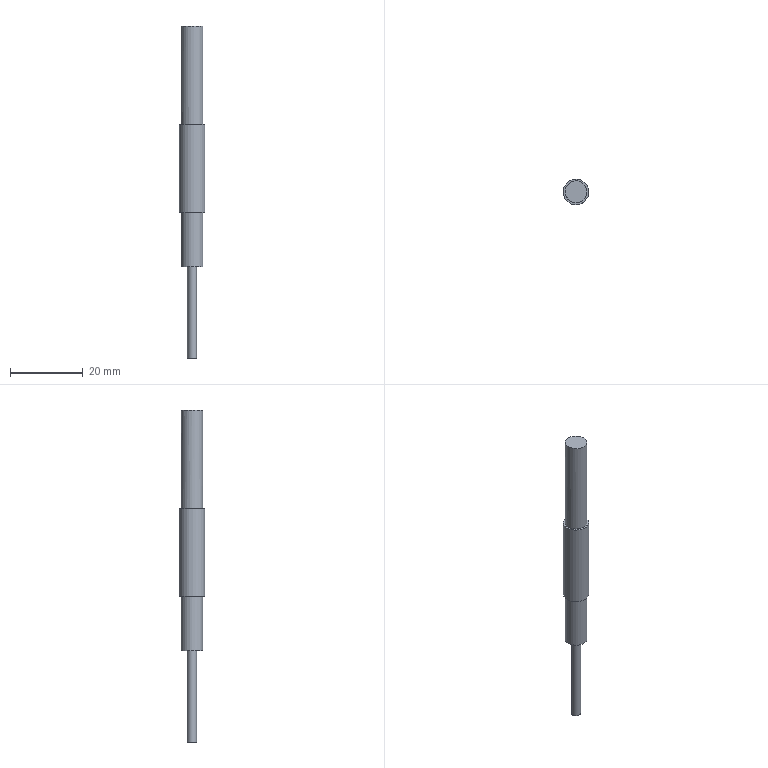Component | NX | DRIVE_SHAFT | 1 solid | 9 faces | box 7 x 7 x 91 mm | volume 2234 mm3 | plane 5 | cylinder 4 | commonest cylinder face diameters 6 x2 7 x1 2.5 x1
STEP:
#1=CARTESIAN_POINT('',(0.,0.,0.));
#2=DIRECTION('',(0.,0.,1.));
#3=DIRECTION('',(1.,0.,0.));
#4=AXIS2_PLACEMENT_3D('',#1,#2,#3);
#5=CARTESIAN_POINT('',(-3.16,-2.811,44.));
#6=VERTEX_POINT('',#5);
#7=CARTESIAN_POINT('',(-5.267,-0.01624,44.));
#8=DIRECTION('',(0.,0.,1.));
#9=DIRECTION('',(0.6018,-0.7986,0.));
#10=AXIS2_PLACEMENT_3D('',#7,#8,#9);
#11=CIRCLE('',#10,3.5);
#12=CARTESIAN_POINT('',(-2.871,1.789,44.));
#13=DIRECTION('',(0.,0.,1.));
#14=DIRECTION('',(0.6018,-0.7986,0.));
#15=AXIS2_PLACEMENT_3D('',#12,#13,#14);
#16=PLANE('',#15);
#17=CARTESIAN_POINT('',(0.,-3.));
#18=DIRECTION('',(1.,0.));
#19=AXIS2_PLACEMENT_2D('',#17,#18);
#20=CIRCLE('',#19,3.5);
#21=(GEOMETRIC_REPRESENTATION_CONTEXT(2)PARAMETRIC_REPRESENTATION_CONTEXT()REPRESENTATION_CONTEXT('',''));
#22=DEFINITIONAL_REPRESENTATION('',(#20),#21);
#23=PCURVE('',#16,#22);
#24=CARTESIAN_POINT('',(-5.267,-0.01624,56.));
#25=DIRECTION('',(0.,0.,1.));
#26=DIRECTION('',(0.6018,-0.7986,0.));
#27=AXIS2_PLACEMENT_3D('',#24,#25,#26);
#28=CYLINDRICAL_SURFACE('',#27,3.5);
#29=CARTESIAN_POINT('',(0.,-12.));
#30=DIRECTION('',(1.,0.));
#31=VECTOR('',#30,1.);
#32=LINE('',#29,#31);
#33=(GEOMETRIC_REPRESENTATION_CONTEXT(2)PARAMETRIC_REPRESENTATION_CONTEXT()REPRESENTATION_CONTEXT('',''));
#34=DEFINITIONAL_REPRESENTATION('',(#32),#33);
#35=PCURVE('',#28,#34);
#36=SURFACE_CURVE('',#11,(#23,#35),.PCURVE_S1.);
#37=EDGE_CURVE('',#6,#6,#36,.T.);
#38=ORIENTED_EDGE('',*,*,#37,.T.);
#39=EDGE_LOOP('',(#38));
#40=FACE_BOUND('',#39,.T.);
#41=CARTESIAN_POINT('',(-3.461,-2.412,44.));
#42=VERTEX_POINT('',#41);
#43=CARTESIAN_POINT('',(-5.267,-0.01624,44.));
#44=DIRECTION('',(0.,0.,1.));
#45=DIRECTION('',(0.6018,-0.7986,0.));
#46=AXIS2_PLACEMENT_3D('',#43,#44,#45);
#47=CIRCLE('',#46,3.);
#48=CARTESIAN_POINT('',(0.,-3.));
#49=DIRECTION('',(1.,0.));
#50=AXIS2_PLACEMENT_2D('',#48,#49);
#51=CIRCLE('',#50,3.);
#52=(GEOMETRIC_REPRESENTATION_CONTEXT(2)PARAMETRIC_REPRESENTATION_CONTEXT()REPRESENTATION_CONTEXT('',''));
#53=DEFINITIONAL_REPRESENTATION('',(#51),#52);
#54=PCURVE('',#16,#53);
#55=CARTESIAN_POINT('',(-5.267,-0.01624,56.));
#56=DIRECTION('',(0.,0.,1.));
#57=DIRECTION('',(0.6018,-0.7986,0.));
#58=AXIS2_PLACEMENT_3D('',#55,#56,#57);
#59=CYLINDRICAL_SURFACE('',#58,3.);
#60=CARTESIAN_POINT('',(0.,-12.));
#61=DIRECTION('',(1.,0.));
#62=VECTOR('',#61,1.);
#63=LINE('',#60,#62);
#64=(GEOMETRIC_REPRESENTATION_CONTEXT(2)PARAMETRIC_REPRESENTATION_CONTEXT()REPRESENTATION_CONTEXT('',''));
#65=DEFINITIONAL_REPRESENTATION('',(#63),#64);
#66=PCURVE('',#59,#65);
#67=SURFACE_CURVE('',#47,(#54,#66),.PCURVE_S1.);
#68=EDGE_CURVE('',#42,#42,#67,.T.);
#69=ORIENTED_EDGE('',*,*,#68,.F.);
#70=EDGE_LOOP('',(#69));
#71=FACE_BOUND('',#70,.T.);
#72=ADVANCED_FACE('',(#40,#71),#16,.T.);
#73=CARTESIAN_POINT('',(-3.16,-2.811,20.));
#74=VERTEX_POINT('',#73);
#75=CARTESIAN_POINT('',(-5.267,-0.01624,20.));
#76=DIRECTION('',(0.,0.,1.));
#77=DIRECTION('',(0.6018,-0.7986,0.));
#78=AXIS2_PLACEMENT_3D('',#75,#76,#77);
#79=CIRCLE('',#78,3.5);
#80=CARTESIAN_POINT('',(0.,-36.));
#81=DIRECTION('',(1.,0.));
#82=VECTOR('',#81,1.);
#83=LINE('',#80,#82);
#84=(GEOMETRIC_REPRESENTATION_CONTEXT(2)PARAMETRIC_REPRESENTATION_CONTEXT()REPRESENTATION_CONTEXT('',''));
#85=DEFINITIONAL_REPRESENTATION('',(#83),#84);
#86=PCURVE('',#28,#85);
#87=CARTESIAN_POINT('',(-2.472,2.09,20.));
#88=DIRECTION('',(0.,0.,-1.));
#89=DIRECTION('',(-0.6018,0.7986,0.));
#90=AXIS2_PLACEMENT_3D('',#87,#88,#89);
#91=PLANE('',#90);
#92=CARTESIAN_POINT('',(-3.5,-3.5));
#93=CARTESIAN_POINT('',(-3.5,2.562));
#94=CARTESIAN_POINT('',(1.75,-0.4689));
#95=CARTESIAN_POINT('',(7.,-3.5));
#96=CARTESIAN_POINT('',(1.75,-6.531));
#97=CARTESIAN_POINT('',(-3.5,-9.562));
#98=CARTESIAN_POINT('',(-3.5,-3.5));
#99=(BOUNDED_CURVE()B_SPLINE_CURVE(2,(#92,#93,#94,#95,#96,#97,#98),.UNSPECIFIED.,.T.,.F.)B_SPLINE_CURVE_WITH_KNOTS((1,2,2,2,2,1),(-2.094,0.,2.094,4.189,6.283,8.378),.UNSPECIFIED.)CURVE()GEOMETRIC_REPRESENTATION_ITEM()RATIONAL_B_SPLINE_CURVE((1.,0.5,1.,0.5,1.,0.5,1.))REPRESENTATION_ITEM(''));
#100=(GEOMETRIC_REPRESENTATION_CONTEXT(2)PARAMETRIC_REPRESENTATION_CONTEXT()REPRESENTATION_CONTEXT('',''));
#101=DEFINITIONAL_REPRESENTATION('',(#99),#100);
#102=PCURVE('',#91,#101);
#103=SURFACE_CURVE('',#79,(#86,#102),.PCURVE_S1.);
#104=EDGE_CURVE('',#74,#74,#103,.T.);
#105=ORIENTED_EDGE('',*,*,#104,.T.);
#106=CARTESIAN_POINT('',(-3.16,-2.811,20.));
#107=CARTESIAN_POINT('',(-3.16,-2.811,44.));
#108=B_SPLINE_CURVE_WITH_KNOTS('',1,(#106,#107),.UNSPECIFIED.,.F.,.F.,(2,2),(-36.,-12.),.PIECEWISE_BEZIER_KNOTS.);
#109=CARTESIAN_POINT('',(6.283,0.));
#110=DIRECTION('',(0.,1.));
#111=VECTOR('',#110,1.);
#112=LINE('',#109,#111);
#113=(GEOMETRIC_REPRESENTATION_CONTEXT(2)PARAMETRIC_REPRESENTATION_CONTEXT()REPRESENTATION_CONTEXT('',''));
#114=DEFINITIONAL_REPRESENTATION('',(#112),#113);
#115=PCURVE('',#28,#114);
#116=CARTESIAN_POINT('',(0.,0.));
#117=DIRECTION('',(0.,1.));
#118=VECTOR('',#117,1.);
#119=LINE('',#116,#118);
#120=(GEOMETRIC_REPRESENTATION_CONTEXT(2)PARAMETRIC_REPRESENTATION_CONTEXT()REPRESENTATION_CONTEXT('',''));
#121=DEFINITIONAL_REPRESENTATION('',(#119),#120);
#122=PCURVE('',#28,#121);
#123=SEAM_CURVE('',#108,(#115,#122),.PCURVE_S1.);
#124=EDGE_CURVE('',#74,#6,#123,.T.);
#125=ORIENTED_EDGE('',*,*,#124,.T.);
#126=ORIENTED_EDGE('',*,*,#37,.F.);
#127=ORIENTED_EDGE('',*,*,#124,.F.);
#128=EDGE_LOOP('',(#105,#125,#126,#127));
#129=FACE_BOUND('',#128,.T.);
#130=ADVANCED_FACE('',(#129),#28,.T.);
#131=CARTESIAN_POINT('',(-3.461,-2.412,20.));
#132=VERTEX_POINT('',#131);
#133=CARTESIAN_POINT('',(-5.267,-0.01624,20.));
#134=DIRECTION('',(0.,0.,1.));
#135=DIRECTION('',(0.6018,-0.7986,0.));
#136=AXIS2_PLACEMENT_3D('',#133,#134,#135);
#137=CIRCLE('',#136,3.);
#138=CARTESIAN_POINT('',(-3.,-3.5));
#139=CARTESIAN_POINT('',(-3.,1.696));
#140=CARTESIAN_POINT('',(1.5,-0.9019));
#141=CARTESIAN_POINT('',(6.,-3.5));
#142=CARTESIAN_POINT('',(1.5,-6.098));
#143=CARTESIAN_POINT('',(-3.,-8.696));
#144=CARTESIAN_POINT('',(-3.,-3.5));
#145=(BOUNDED_CURVE()B_SPLINE_CURVE(2,(#138,#139,#140,#141,#142,#143,#144),.UNSPECIFIED.,.T.,.F.)B_SPLINE_CURVE_WITH_KNOTS((1,2,2,2,2,1),(-2.094,0.,2.094,4.189,6.283,8.378),.UNSPECIFIED.)CURVE()GEOMETRIC_REPRESENTATION_ITEM()RATIONAL_B_SPLINE_CURVE((1.,0.5,1.,0.5,1.,0.5,1.))REPRESENTATION_ITEM(''));
#146=(GEOMETRIC_REPRESENTATION_CONTEXT(2)PARAMETRIC_REPRESENTATION_CONTEXT()REPRESENTATION_CONTEXT('',''));
#147=DEFINITIONAL_REPRESENTATION('',(#145),#146);
#148=PCURVE('',#91,#147);
#149=CARTESIAN_POINT('',(-5.267,-0.01624,56.));
#150=DIRECTION('',(0.,0.,1.));
#151=DIRECTION('',(0.6018,-0.7986,0.));
#152=AXIS2_PLACEMENT_3D('',#149,#150,#151);
#153=CYLINDRICAL_SURFACE('',#152,3.);
#154=CARTESIAN_POINT('',(0.,-36.));
#155=DIRECTION('',(1.,0.));
#156=VECTOR('',#155,1.);
#157=LINE('',#154,#156);
#158=(GEOMETRIC_REPRESENTATION_CONTEXT(2)PARAMETRIC_REPRESENTATION_CONTEXT()REPRESENTATION_CONTEXT('',''));
#159=DEFINITIONAL_REPRESENTATION('',(#157),#158);
#160=PCURVE('',#153,#159);
#161=SURFACE_CURVE('',#137,(#148,#160),.PCURVE_S1.);
#162=EDGE_CURVE('',#132,#132,#161,.T.);
#163=ORIENTED_EDGE('',*,*,#162,.T.);
#164=EDGE_LOOP('',(#163));
#165=FACE_BOUND('',#164,.T.);
#166=ORIENTED_EDGE('',*,*,#104,.F.);
#167=EDGE_LOOP('',(#166));
#168=FACE_BOUND('',#167,.T.);
#169=ADVANCED_FACE('',(#165,#168),#91,.T.);
#170=ORIENTED_EDGE('',*,*,#162,.F.);
#171=CARTESIAN_POINT('',(-3.461,-2.412,5.));
#172=VERTEX_POINT('',#171);
#173=CARTESIAN_POINT('',(-3.461,-2.412,5.));
#174=CARTESIAN_POINT('',(-3.461,-2.412,20.));
#175=B_SPLINE_CURVE_WITH_KNOTS('',1,(#173,#174),.UNSPECIFIED.,.F.,.F.,(2,2),(-51.,-36.),.PIECEWISE_BEZIER_KNOTS.);
#176=CARTESIAN_POINT('',(0.,0.));
#177=DIRECTION('',(0.,1.));
#178=VECTOR('',#177,1.);
#179=LINE('',#176,#178);
#180=(GEOMETRIC_REPRESENTATION_CONTEXT(2)PARAMETRIC_REPRESENTATION_CONTEXT()REPRESENTATION_CONTEXT('',''));
#181=DEFINITIONAL_REPRESENTATION('',(#179),#180);
#182=PCURVE('',#153,#181);
#183=CARTESIAN_POINT('',(6.283,0.));
#184=DIRECTION('',(0.,1.));
#185=VECTOR('',#184,1.);
#186=LINE('',#183,#185);
#187=(GEOMETRIC_REPRESENTATION_CONTEXT(2)PARAMETRIC_REPRESENTATION_CONTEXT()REPRESENTATION_CONTEXT('',''));
#188=DEFINITIONAL_REPRESENTATION('',(#186),#187);
#189=PCURVE('',#153,#188);
#190=SEAM_CURVE('',#175,(#182,#189),.PCURVE_S1.);
#191=EDGE_CURVE('',#172,#132,#190,.T.);
#192=ORIENTED_EDGE('',*,*,#191,.F.);
#193=CARTESIAN_POINT('',(-5.267,-0.01624,5.));
#194=DIRECTION('',(0.,0.,-1.));
#195=DIRECTION('',(0.6018,-0.7986,0.));
#196=AXIS2_PLACEMENT_3D('',#193,#194,#195);
#197=CIRCLE('',#196,3.);
#198=CARTESIAN_POINT('',(6.283,-51.));
#199=DIRECTION('',(-1.,0.));
#200=VECTOR('',#199,1.);
#201=LINE('',#198,#200);
#202=(GEOMETRIC_REPRESENTATION_CONTEXT(2)PARAMETRIC_REPRESENTATION_CONTEXT()REPRESENTATION_CONTEXT('',''));
#203=DEFINITIONAL_REPRESENTATION('',(#201),#202);
#204=PCURVE('',#153,#203);
#205=CARTESIAN_POINT('',(-5.267,-0.01624,5.));
#206=DIRECTION('',(0.,0.,-1.));
#207=DIRECTION('',(-0.6018,0.7986,0.));
#208=AXIS2_PLACEMENT_3D('',#205,#206,#207);
#209=PLANE('',#208);
#210=CARTESIAN_POINT('',(0.,0.));
#211=DIRECTION('',(-1.,0.));
#212=AXIS2_PLACEMENT_2D('',#210,#211);
#213=CIRCLE('',#212,3.);
#214=(GEOMETRIC_REPRESENTATION_CONTEXT(2)PARAMETRIC_REPRESENTATION_CONTEXT()REPRESENTATION_CONTEXT('',''));
#215=DEFINITIONAL_REPRESENTATION('',(#213),#214);
#216=PCURVE('',#209,#215);
#217=SURFACE_CURVE('',#197,(#204,#216),.PCURVE_S1.);
#218=EDGE_CURVE('',#172,#172,#217,.T.);
#219=ORIENTED_EDGE('',*,*,#218,.F.);
#220=ORIENTED_EDGE('',*,*,#191,.T.);
#221=EDGE_LOOP('',(#170,#192,#219,#220));
#222=FACE_BOUND('',#221,.T.);
#223=ADVANCED_FACE('',(#222),#153,.T.);
#224=ORIENTED_EDGE('',*,*,#68,.T.);
#225=CARTESIAN_POINT('',(-3.461,-2.412,71.));
#226=VERTEX_POINT('',#225);
#227=CARTESIAN_POINT('',(-3.461,-2.412,44.));
#228=CARTESIAN_POINT('',(-3.461,-2.412,71.));
#229=B_SPLINE_CURVE_WITH_KNOTS('',1,(#227,#228),.UNSPECIFIED.,.F.,.F.,(2,2),(-12.,15.),.PIECEWISE_BEZIER_KNOTS.);
#230=CARTESIAN_POINT('',(6.283,0.));
#231=DIRECTION('',(0.,1.));
#232=VECTOR('',#231,1.);
#233=LINE('',#230,#232);
#234=(GEOMETRIC_REPRESENTATION_CONTEXT(2)PARAMETRIC_REPRESENTATION_CONTEXT()REPRESENTATION_CONTEXT('',''));
#235=DEFINITIONAL_REPRESENTATION('',(#233),#234);
#236=PCURVE('',#59,#235);
#237=CARTESIAN_POINT('',(0.,0.));
#238=DIRECTION('',(0.,1.));
#239=VECTOR('',#238,1.);
#240=LINE('',#237,#239);
#241=(GEOMETRIC_REPRESENTATION_CONTEXT(2)PARAMETRIC_REPRESENTATION_CONTEXT()REPRESENTATION_CONTEXT('',''));
#242=DEFINITIONAL_REPRESENTATION('',(#240),#241);
#243=PCURVE('',#59,#242);
#244=SEAM_CURVE('',#229,(#236,#243),.PCURVE_S1.);
#245=EDGE_CURVE('',#42,#226,#244,.T.);
#246=ORIENTED_EDGE('',*,*,#245,.T.);
#247=CARTESIAN_POINT('',(-2.871,1.789,71.));
#248=VERTEX_POINT('',#247);
#249=CARTESIAN_POINT('',(-5.267,-0.01624,71.));
#250=DIRECTION('',(0.,0.,-1.));
#251=DIRECTION('',(0.7986,0.6018,0.));
#252=AXIS2_PLACEMENT_3D('',#249,#250,#251);
#253=CIRCLE('',#252,3.);
#254=CARTESIAN_POINT('',(7.854,15.));
#255=DIRECTION('',(-1.,0.));
#256=VECTOR('',#255,1.);
#257=LINE('',#254,#256);
#258=(GEOMETRIC_REPRESENTATION_CONTEXT(2)PARAMETRIC_REPRESENTATION_CONTEXT()REPRESENTATION_CONTEXT('',''));
#259=DEFINITIONAL_REPRESENTATION('',(#257),#258);
#260=PCURVE('',#59,#259);
#261=CARTESIAN_POINT('',(-5.267,-0.01624,71.));
#262=DIRECTION('',(0.,0.,-1.));
#263=DIRECTION('',(-0.6018,0.7986,0.));
#264=AXIS2_PLACEMENT_3D('',#261,#262,#263);
#265=PLANE('',#264);
#266=CARTESIAN_POINT('',(0.,0.));
#267=DIRECTION('',(0.,1.));
#268=AXIS2_PLACEMENT_2D('',#266,#267);
#269=CIRCLE('',#268,3.);
#270=(GEOMETRIC_REPRESENTATION_CONTEXT(2)PARAMETRIC_REPRESENTATION_CONTEXT()REPRESENTATION_CONTEXT('',''));
#271=DEFINITIONAL_REPRESENTATION('',(#269),#270);
#272=PCURVE('',#265,#271);
#273=SURFACE_CURVE('',#253,(#260,#272),.PCURVE_S1.);
#274=EDGE_CURVE('',#226,#248,#273,.T.);
#275=ORIENTED_EDGE('',*,*,#274,.T.);
#276=CARTESIAN_POINT('',(-5.267,-0.01624,71.));
#277=DIRECTION('',(0.,0.,-1.));
#278=DIRECTION('',(0.7986,0.6018,0.));
#279=AXIS2_PLACEMENT_3D('',#276,#277,#278);
#280=CIRCLE('',#279,3.);
#281=CARTESIAN_POINT('',(1.571,15.));
#282=DIRECTION('',(-1.,0.));
#283=VECTOR('',#282,1.);
#284=LINE('',#281,#283);
#285=(GEOMETRIC_REPRESENTATION_CONTEXT(2)PARAMETRIC_REPRESENTATION_CONTEXT()REPRESENTATION_CONTEXT('',''));
#286=DEFINITIONAL_REPRESENTATION('',(#284),#285);
#287=PCURVE('',#59,#286);
#288=CARTESIAN_POINT('',(0.,0.));
#289=DIRECTION('',(0.,1.));
#290=AXIS2_PLACEMENT_2D('',#288,#289);
#291=CIRCLE('',#290,3.);
#292=(GEOMETRIC_REPRESENTATION_CONTEXT(2)PARAMETRIC_REPRESENTATION_CONTEXT()REPRESENTATION_CONTEXT('',''));
#293=DEFINITIONAL_REPRESENTATION('',(#291),#292);
#294=PCURVE('',#265,#293);
#295=SURFACE_CURVE('',#280,(#287,#294),.PCURVE_S1.);
#296=EDGE_CURVE('',#248,#226,#295,.T.);
#297=ORIENTED_EDGE('',*,*,#296,.T.);
#298=ORIENTED_EDGE('',*,*,#245,.F.);
#299=EDGE_LOOP('',(#224,#246,#275,#297,#298));
#300=FACE_BOUND('',#299,.T.);
#301=ADVANCED_FACE('',(#300),#59,.T.);
#302=CARTESIAN_POINT('',(-6.019,0.9821,5.));
#303=VERTEX_POINT('',#302);
#304=CARTESIAN_POINT('',(-4.514,-1.015,5.));
#305=VERTEX_POINT('',#304);
#306=CARTESIAN_POINT('',(-5.267,-0.01624,5.));
#307=DIRECTION('',(0.,0.,1.));
#308=DIRECTION('',(-0.6018,0.7986,0.));
#309=AXIS2_PLACEMENT_3D('',#306,#307,#308);
#310=CIRCLE('',#309,1.25);
#311=CARTESIAN_POINT('',(1.25,0.));
#312=CARTESIAN_POINT('',(1.25,-2.165));
#313=CARTESIAN_POINT('',(-0.625,-1.083));
#314=CARTESIAN_POINT('',(-2.5,-0.));
#315=CARTESIAN_POINT('',(-0.625,1.083));
#316=CARTESIAN_POINT('',(1.25,2.165));
#317=CARTESIAN_POINT('',(1.25,0.));
#318=(BOUNDED_CURVE()B_SPLINE_CURVE(2,(#311,#312,#313,#314,#315,#316,#317),.UNSPECIFIED.,.T.,.F.)B_SPLINE_CURVE_WITH_KNOTS((1,2,2,2,2,1),(-2.094,0.,2.094,4.189,6.283,8.378),.UNSPECIFIED.)CURVE()GEOMETRIC_REPRESENTATION_ITEM()RATIONAL_B_SPLINE_CURVE((1.,0.5,1.,0.5,1.,0.5,1.))REPRESENTATION_ITEM(''));
#319=(GEOMETRIC_REPRESENTATION_CONTEXT(2)PARAMETRIC_REPRESENTATION_CONTEXT()REPRESENTATION_CONTEXT('',''));
#320=DEFINITIONAL_REPRESENTATION('',(#318),#319);
#321=PCURVE('',#209,#320);
#322=CARTESIAN_POINT('',(-5.267,-0.01624,56.));
#323=DIRECTION('',(0.,0.,1.));
#324=DIRECTION('',(0.6018,-0.7986,0.));
#325=AXIS2_PLACEMENT_3D('',#322,#323,#324);
#326=CYLINDRICAL_SURFACE('',#325,1.25);
#327=CARTESIAN_POINT('',(3.142,-51.));
#328=DIRECTION('',(1.,0.));
#329=VECTOR('',#328,1.);
#330=LINE('',#327,#329);
#331=(GEOMETRIC_REPRESENTATION_CONTEXT(2)PARAMETRIC_REPRESENTATION_CONTEXT()REPRESENTATION_CONTEXT('',''));
#332=DEFINITIONAL_REPRESENTATION('',(#330),#331);
#333=PCURVE('',#326,#332);
#334=SURFACE_CURVE('',#310,(#321,#333),.PCURVE_S1.);
#335=EDGE_CURVE('',#303,#305,#334,.T.);
#336=ORIENTED_EDGE('',*,*,#335,.T.);
#337=CARTESIAN_POINT('',(-5.267,-0.01624,5.));
#338=DIRECTION('',(0.,0.,1.));
#339=DIRECTION('',(-0.6018,0.7986,0.));
#340=AXIS2_PLACEMENT_3D('',#337,#338,#339);
#341=CIRCLE('',#340,1.25);
#342=CARTESIAN_POINT('',(1.25,0.));
#343=CARTESIAN_POINT('',(1.25,-2.165));
#344=CARTESIAN_POINT('',(-0.625,-1.083));
#345=CARTESIAN_POINT('',(-2.5,-0.));
#346=CARTESIAN_POINT('',(-0.625,1.083));
#347=CARTESIAN_POINT('',(1.25,2.165));
#348=CARTESIAN_POINT('',(1.25,0.));
#349=(BOUNDED_CURVE()B_SPLINE_CURVE(2,(#342,#343,#344,#345,#346,#347,#348),.UNSPECIFIED.,.T.,.F.)B_SPLINE_CURVE_WITH_KNOTS((1,2,2,2,2,1),(-2.094,0.,2.094,4.189,6.283,8.378),.UNSPECIFIED.)CURVE()GEOMETRIC_REPRESENTATION_ITEM()RATIONAL_B_SPLINE_CURVE((1.,0.5,1.,0.5,1.,0.5,1.))REPRESENTATION_ITEM(''));
#350=(GEOMETRIC_REPRESENTATION_CONTEXT(2)PARAMETRIC_REPRESENTATION_CONTEXT()REPRESENTATION_CONTEXT('',''));
#351=DEFINITIONAL_REPRESENTATION('',(#349),#350);
#352=PCURVE('',#209,#351);
#353=CARTESIAN_POINT('',(-3.142,-51.));
#354=DIRECTION('',(1.,0.));
#355=VECTOR('',#354,1.);
#356=LINE('',#353,#355);
#357=(GEOMETRIC_REPRESENTATION_CONTEXT(2)PARAMETRIC_REPRESENTATION_CONTEXT()REPRESENTATION_CONTEXT('',''));
#358=DEFINITIONAL_REPRESENTATION('',(#356),#357);
#359=PCURVE('',#326,#358);
#360=SURFACE_CURVE('',#341,(#352,#359),.PCURVE_S1.);
#361=EDGE_CURVE('',#305,#303,#360,.T.);
#362=ORIENTED_EDGE('',*,*,#361,.T.);
#363=EDGE_LOOP('',(#336,#362));
#364=FACE_BOUND('',#363,.T.);
#365=ORIENTED_EDGE('',*,*,#218,.T.);
#366=EDGE_LOOP('',(#365));
#367=FACE_BOUND('',#366,.T.);
#368=ADVANCED_FACE('',(#364,#367),#209,.T.);
#369=CARTESIAN_POINT('',(-4.514,-1.015,-20.));
#370=VERTEX_POINT('',#369);
#371=CARTESIAN_POINT('',(-5.267,-0.01624,-20.));
#372=DIRECTION('',(0.,0.,1.));
#373=DIRECTION('',(0.6018,-0.7986,0.));
#374=AXIS2_PLACEMENT_3D('',#371,#372,#373);
#375=CIRCLE('',#374,1.25);
#376=CARTESIAN_POINT('',(-4.268,0.736,-20.));
#377=DIRECTION('',(0.,0.,-1.));
#378=DIRECTION('',(-0.6018,0.7986,0.));
#379=AXIS2_PLACEMENT_3D('',#376,#377,#378);
#380=PLANE('',#379);
#381=CARTESIAN_POINT('',(-1.25,-1.25));
#382=CARTESIAN_POINT('',(-1.25,0.9151));
#383=CARTESIAN_POINT('',(0.625,-0.1675));
#384=CARTESIAN_POINT('',(2.5,-1.25));
#385=CARTESIAN_POINT('',(0.625,-2.333));
#386=CARTESIAN_POINT('',(-1.25,-3.415));
#387=CARTESIAN_POINT('',(-1.25,-1.25));
#388=(BOUNDED_CURVE()B_SPLINE_CURVE(2,(#381,#382,#383,#384,#385,#386,#387),.UNSPECIFIED.,.T.,.F.)B_SPLINE_CURVE_WITH_KNOTS((1,2,2,2,2,1),(-2.094,0.,2.094,4.189,6.283,8.378),.UNSPECIFIED.)CURVE()GEOMETRIC_REPRESENTATION_ITEM()RATIONAL_B_SPLINE_CURVE((1.,0.5,1.,0.5,1.,0.5,1.))REPRESENTATION_ITEM(''));
#389=(GEOMETRIC_REPRESENTATION_CONTEXT(2)PARAMETRIC_REPRESENTATION_CONTEXT()REPRESENTATION_CONTEXT('',''));
#390=DEFINITIONAL_REPRESENTATION('',(#388),#389);
#391=PCURVE('',#380,#390);
#392=CARTESIAN_POINT('',(0.,-76.));
#393=DIRECTION('',(1.,0.));
#394=VECTOR('',#393,1.);
#395=LINE('',#392,#394);
#396=(GEOMETRIC_REPRESENTATION_CONTEXT(2)PARAMETRIC_REPRESENTATION_CONTEXT()REPRESENTATION_CONTEXT('',''));
#397=DEFINITIONAL_REPRESENTATION('',(#395),#396);
#398=PCURVE('',#326,#397);
#399=SURFACE_CURVE('',#375,(#391,#398),.PCURVE_S1.);
#400=EDGE_CURVE('',#370,#370,#399,.T.);
#401=ORIENTED_EDGE('',*,*,#400,.F.);
#402=EDGE_LOOP('',(#401));
#403=FACE_BOUND('',#402,.T.);
#404=ADVANCED_FACE('',(#403),#380,.T.);
#405=ORIENTED_EDGE('',*,*,#361,.F.);
#406=CARTESIAN_POINT('',(-4.514,-1.015,-20.));
#407=CARTESIAN_POINT('',(-4.514,-1.015,5.));
#408=B_SPLINE_CURVE_WITH_KNOTS('',1,(#406,#407),.UNSPECIFIED.,.F.,.F.,(2,2),(-76.,-51.),.PIECEWISE_BEZIER_KNOTS.);
#409=CARTESIAN_POINT('',(0.,0.));
#410=DIRECTION('',(0.,1.));
#411=VECTOR('',#410,1.);
#412=LINE('',#409,#411);
#413=(GEOMETRIC_REPRESENTATION_CONTEXT(2)PARAMETRIC_REPRESENTATION_CONTEXT()REPRESENTATION_CONTEXT('',''));
#414=DEFINITIONAL_REPRESENTATION('',(#412),#413);
#415=PCURVE('',#326,#414);
#416=CARTESIAN_POINT('',(6.283,0.));
#417=DIRECTION('',(0.,1.));
#418=VECTOR('',#417,1.);
#419=LINE('',#416,#418);
#420=(GEOMETRIC_REPRESENTATION_CONTEXT(2)PARAMETRIC_REPRESENTATION_CONTEXT()REPRESENTATION_CONTEXT('',''));
#421=DEFINITIONAL_REPRESENTATION('',(#419),#420);
#422=PCURVE('',#326,#421);
#423=SEAM_CURVE('',#408,(#415,#422),.PCURVE_S1.);
#424=EDGE_CURVE('',#370,#305,#423,.T.);
#425=ORIENTED_EDGE('',*,*,#424,.F.);
#426=ORIENTED_EDGE('',*,*,#400,.T.);
#427=ORIENTED_EDGE('',*,*,#424,.T.);
#428=ORIENTED_EDGE('',*,*,#335,.F.);
#429=EDGE_LOOP('',(#405,#425,#426,#427,#428));
#430=FACE_BOUND('',#429,.T.);
#431=ADVANCED_FACE('',(#430),#326,.T.);
#432=ORIENTED_EDGE('',*,*,#296,.F.);
#433=ORIENTED_EDGE('',*,*,#274,.F.);
#434=EDGE_LOOP('',(#432,#433));
#435=FACE_BOUND('',#434,.T.);
#436=ADVANCED_FACE('',(#435),#265,.F.);
#437=CLOSED_SHELL('',(#72,#130,#169,#223,#301,#368,#404,#431,#436));
#438=MANIFOLD_SOLID_BREP('',#437);
#439=(LENGTH_UNIT()NAMED_UNIT(*)SI_UNIT(.MILLI.,.METRE.));
#440=UNCERTAINTY_MEASURE_WITH_UNIT(LENGTH_MEASURE(0.000005),#439,'','');
#441=(NAMED_UNIT(*)PLANE_ANGLE_UNIT()SI_UNIT($,.RADIAN.));
#442=(NAMED_UNIT(*)SI_UNIT($,.STERADIAN.)SOLID_ANGLE_UNIT());
#443=(GEOMETRIC_REPRESENTATION_CONTEXT(3)GLOBAL_UNCERTAINTY_ASSIGNED_CONTEXT((#440))GLOBAL_UNIT_ASSIGNED_CONTEXT((#439,#441,#442))REPRESENTATION_CONTEXT('',''));
#444=ADVANCED_BREP_SHAPE_REPRESENTATION('',(#4,#438),#443);